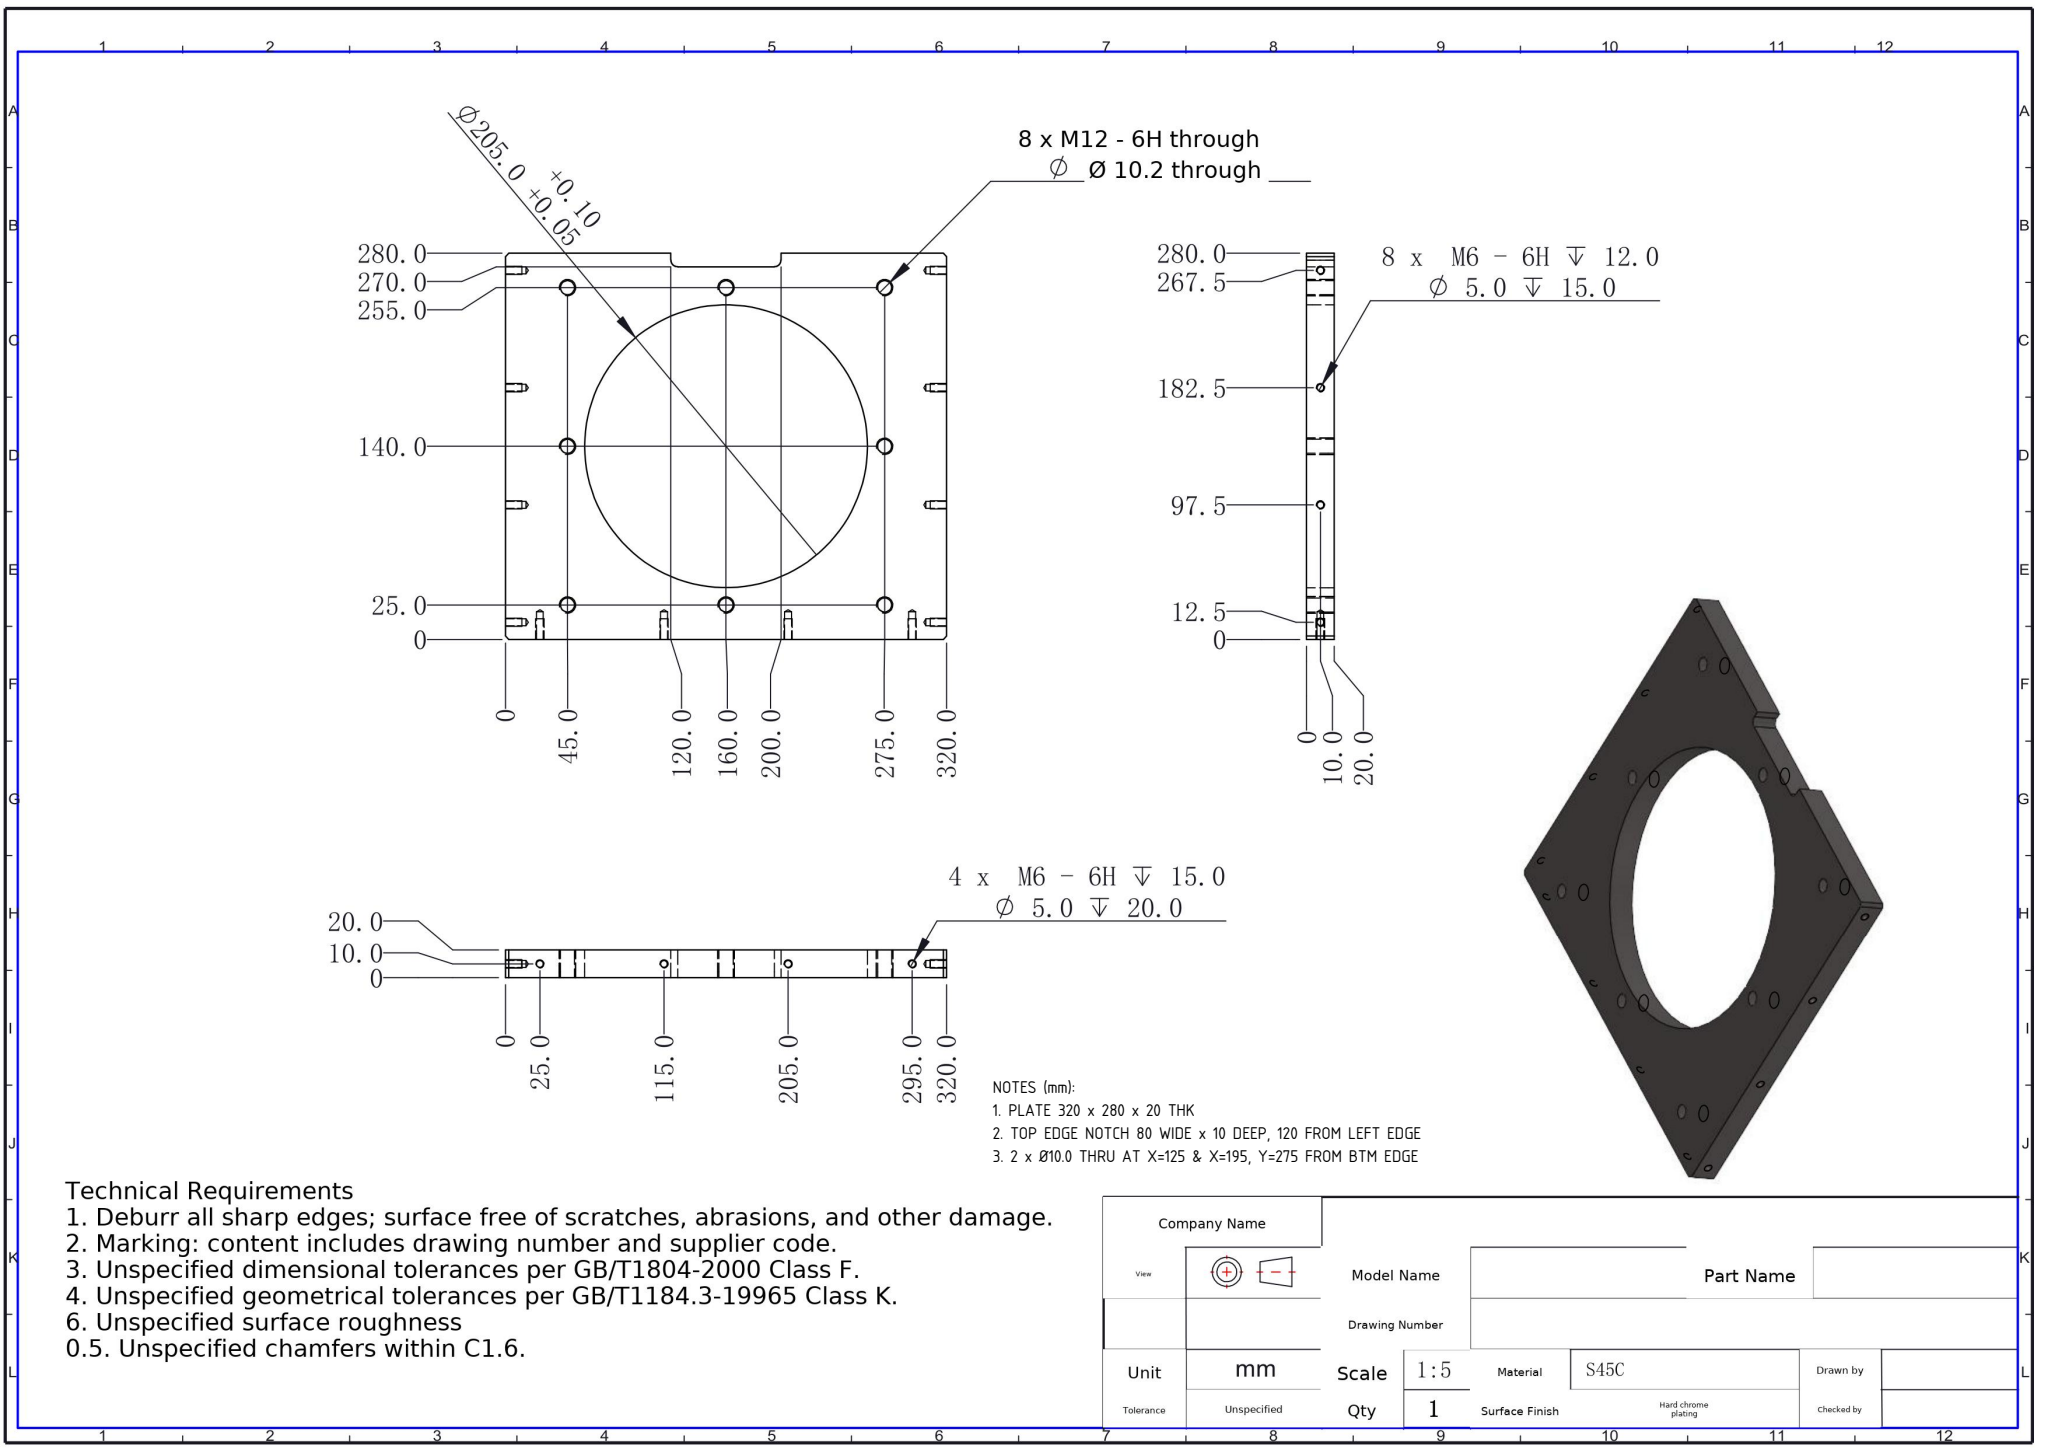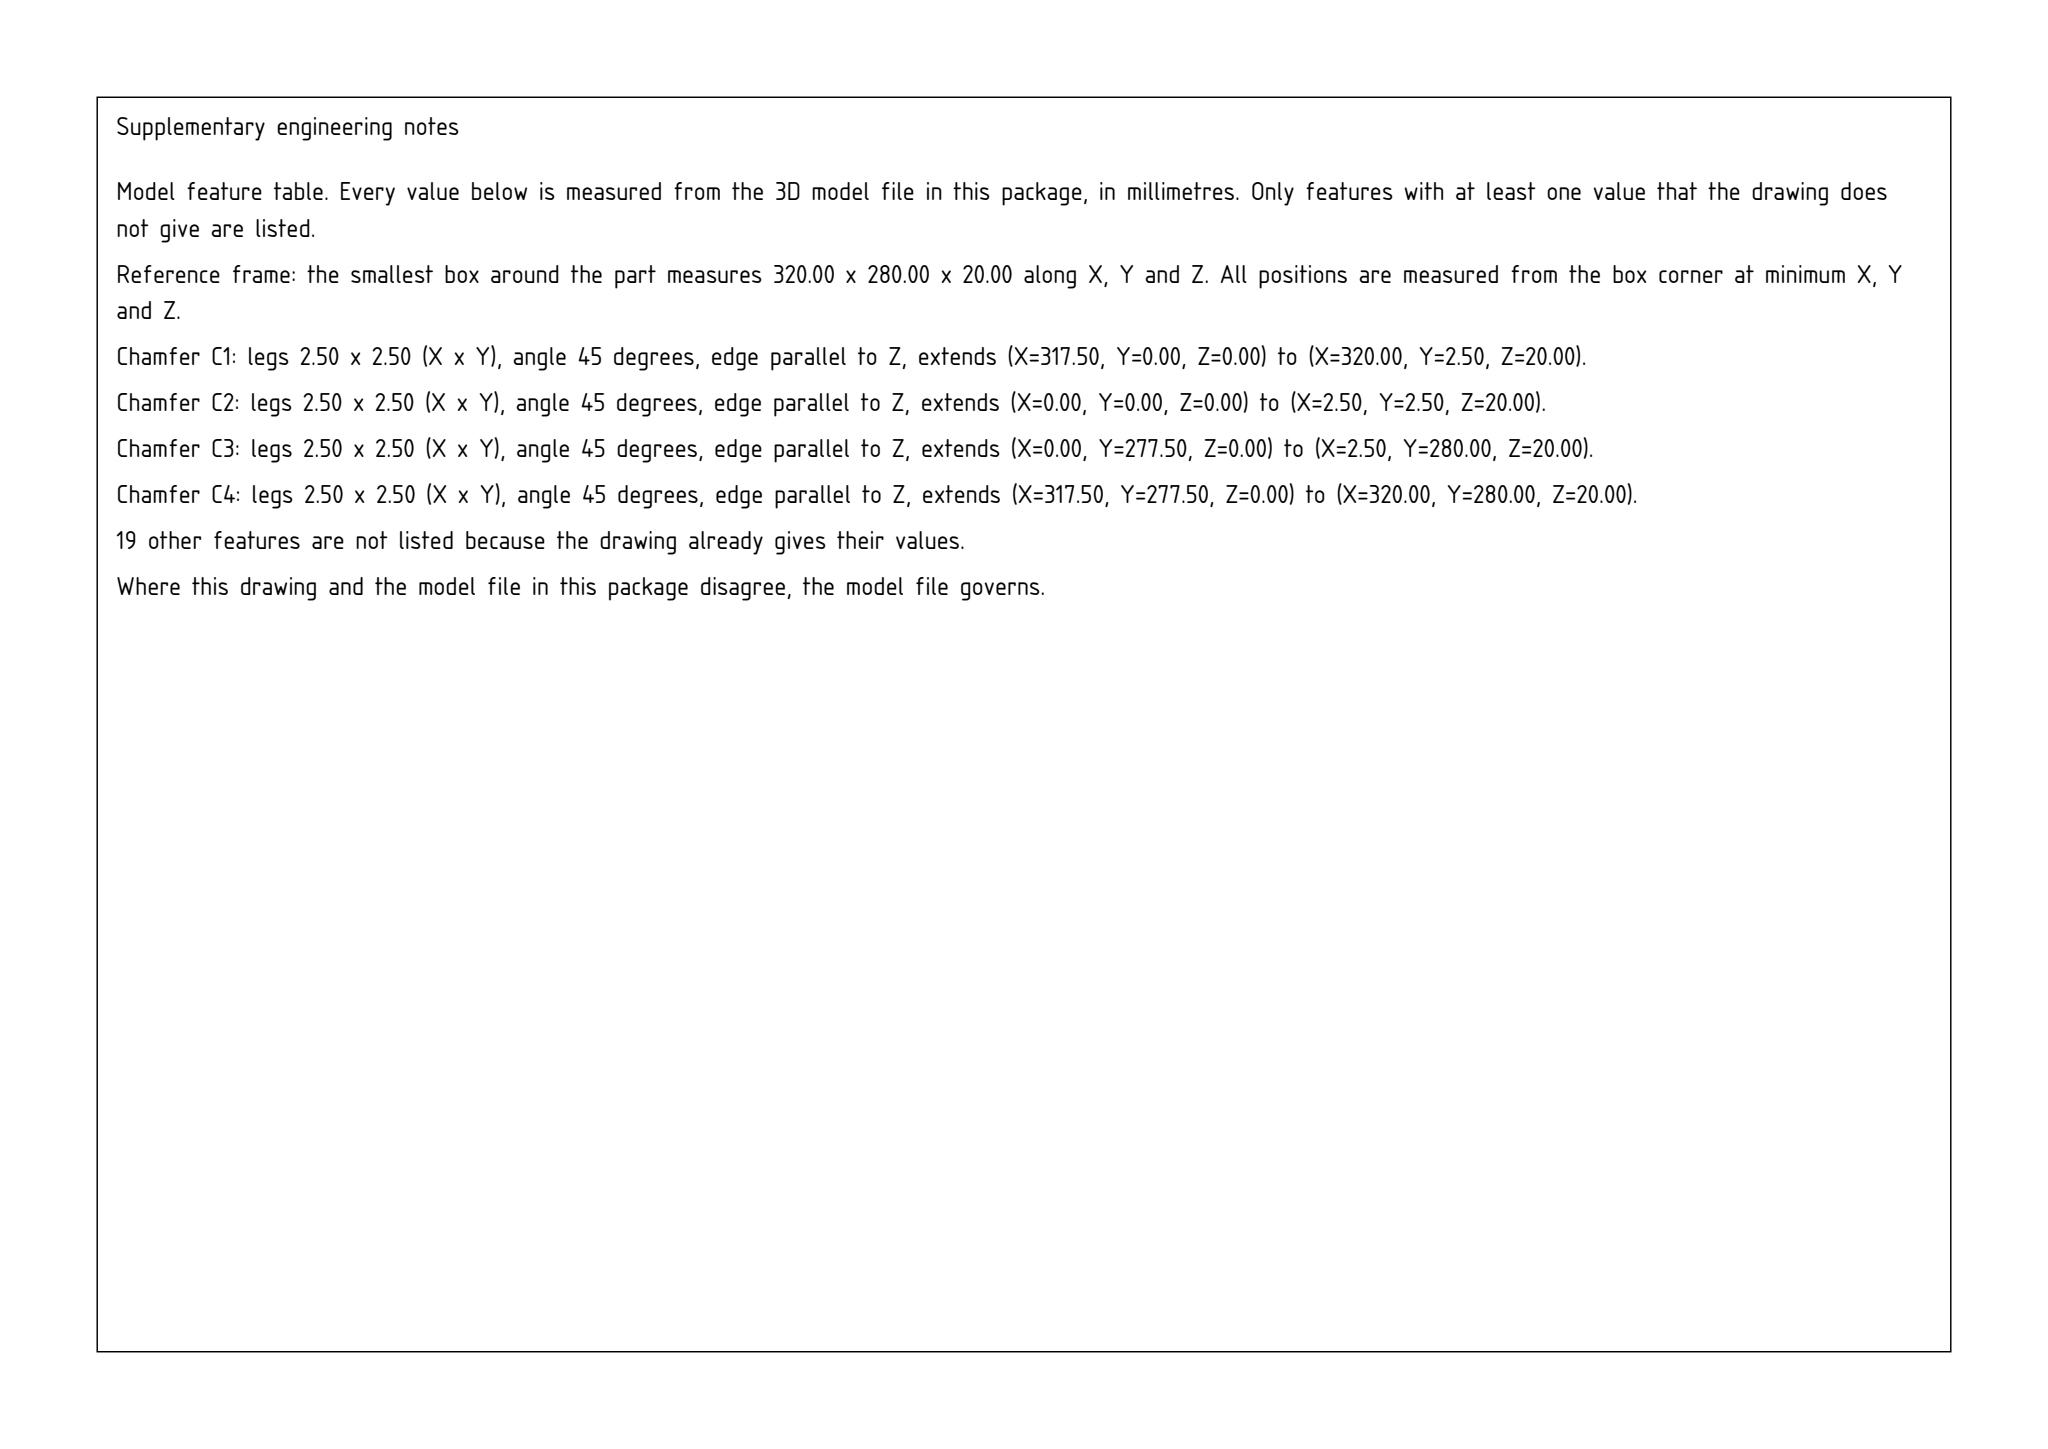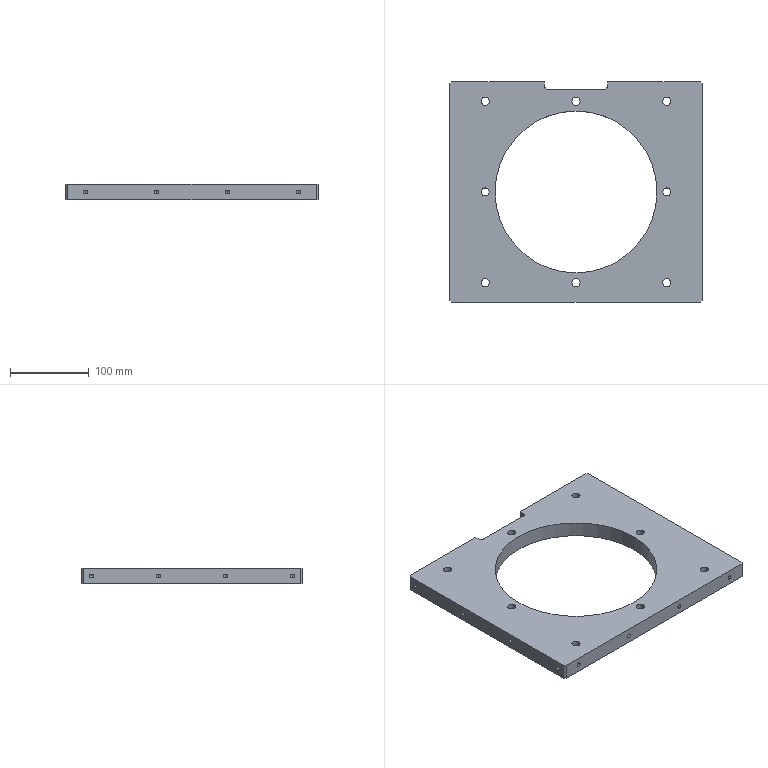Part | SolidWorks | mm | 1 solid | 82 faces | box 320 x 280 x 20 mm | volume 1098718 mm3 | cylinder 44 | cone 24 | plane 14 | commonest cylinder face diameters 5 x24 10.2 x16 205 x2 10 x2
Drawing notes:
PLATE 320 x 280 x 20 THK | from the solid: bbox_xyz 320.0 x 280.0 x 20.0
TOP EDGE NOTCH 80 WIDE x 10 DEEP, 120 FROM LEFT EDGE | from the solid: x planes 120.0 & 200.0 with y plane 270.0 vs top face y=280.0; 200-120=80, 280-270=10
2 x Ø10.0 THRU AT X=125 & X=195, Y=275 FROM BTM EDGE | from the solid: cylinders dia 10.0 axis z at (125,275) and (195,275), length 20 = full plate thk
build123d program:
from build123d import *

# Parameters (mm, degrees)
SKETCH1_R                  = 102.5
BOSS_EXTRUDE1_DEPTH        = 10
M6_TAPPED_HOLE1_AT_2_COUNT = 2
M6_TAPPED_HOLE1_AT_2_PITCH = 85
M6_TAPPED_HOLE1_AT_3_COUNT = 2
M6_TAPPED_HOLE1_AT_3_PITCH = 170
M6_TAPPED_HOLE1_AT_4_COUNT = 2
M6_TAPPED_HOLE1_AT_4_PITCH = 255
M12_TAPPED_HOLE1_D         = 10.2
M6_TAPPED_HOLE2_D          = 5
M6_TAPPED_HOLE2_DEPTH      = 20
M6_TAPPED_HOLE2_TIP        = 1.502
CHAMFER1_SIZE              = 2.5
FILLET1_R                  = 5


with BuildPart() as part:
    # Sketch1 → Boss-Extrude1 (new, symmetric)
    with BuildSketch(Plane.XY):
        Polygon((-160, 140), (-40, 140), (-40, 130), (40, 130), (40, 140), (160, 140), (160, -140), (-160, -140), align=None)
        Circle(SKETCH1_R, mode=Mode.SUBTRACT)
    extrude(amount=BOSS_EXTRUDE1_DEPTH, both=True)

    # Sketch3 → M6 Tapped Hole1 (revolve, cut)
    with BuildSketch(Plane(origin=(160, 127.5, 0), x_dir=(0, 0, -1), z_dir=(0, 1, 0))):
        Polygon((0, 0), (0, 16.502), (2.5, 15), (2.5, 0), align=None)
    m6_tapped_hole1 = revolve(axis=Axis((166.35, 127.5, 0), (-1, 0, 0)), mode=Mode.SUBTRACT)

    # M6 Tapped Hole1 at 2: M6 Tapped Hole1 ×2
    with Locations(*[(0, -i * M6_TAPPED_HOLE1_AT_2_PITCH, 0) for i in range(1, M6_TAPPED_HOLE1_AT_2_COUNT)]):
        add(m6_tapped_hole1, mode=Mode.SUBTRACT)

    # M6 Tapped Hole1 at 3: M6 Tapped Hole1 ×2
    with Locations(*[(0, -i * M6_TAPPED_HOLE1_AT_3_PITCH, 0) for i in range(1, M6_TAPPED_HOLE1_AT_3_COUNT)]):
        add(m6_tapped_hole1, mode=Mode.SUBTRACT)

    # M6 Tapped Hole1 at 4: M6 Tapped Hole1 ×2
    with Locations(*[(0, -i * M6_TAPPED_HOLE1_AT_4_PITCH, 0) for i in range(1, M6_TAPPED_HOLE1_AT_4_COUNT)]):
        add(m6_tapped_hole1, mode=Mode.SUBTRACT)

    # Mirror1: M6 Tapped Hole1 across plane
    add(m6_tapped_hole1.mirror(Plane(origin=(0, 0, 0), x_dir=(0, 0, 1), z_dir=(1, 0, 0))), mode=Mode.SUBTRACT)

    # Mirror1 copy 1 sketch → Mirror1 copy 1 (revolve, cut)
    with BuildSketch(Plane(origin=(-160, 42.5, 0), x_dir=(0, 0, -1), z_dir=(0, 1, 0))):
        Polygon((0, 0), (0, -16.502), (2.5, -15), (2.5, 0), align=None)
    revolve(axis=Axis((-166.35, 42.5, 0), (-1, 0, 0)), mode=Mode.SUBTRACT)

    # Mirror1 copy 2 sketch → Mirror1 copy 2 (revolve, cut)
    with BuildSketch(Plane(origin=(-160, -42.5, 0), x_dir=(0, 0, -1), z_dir=(0, 1, 0))):
        Polygon((0, 0), (0, -16.502), (2.5, -15), (2.5, 0), align=None)
    revolve(axis=Axis((-166.35, -42.5, 0), (-1, 0, 0)), mode=Mode.SUBTRACT)

    # Mirror1 copy 3 sketch → Mirror1 copy 3 (revolve, cut)
    with BuildSketch(Plane(origin=(-160, -127.5, 0), x_dir=(0, 0, -1), z_dir=(0, 1, 0))):
        Polygon((0, 0), (0, -16.502), (2.5, -15), (2.5, 0), align=None)
    revolve(axis=Axis((-166.35, -127.5, 0), (-1, 0, 0)), mode=Mode.SUBTRACT)

    # M12 Tapped Hole1 (through all)
    with Locations(Plane.XY.offset(10)):
        with Locations((-115, 115), (-115, 0), (0, 115), (115, 115), (115, 0), (115, -115), (0, -115), (-115, -115)):
            Hole(M12_TAPPED_HOLE1_D / 2)

    # M6 Tapped Hole2
    with Locations(Plane(origin=(0, -140, 0), x_dir=(-1, 0, 0), z_dir=(0, -1, 0))):
        with Locations((-135, 0), (-45, 0), (45, 0), (135, 0)):
            Hole(M6_TAPPED_HOLE2_D / 2, depth=M6_TAPPED_HOLE2_DEPTH)
            with Locations((0, 0, -(M6_TAPPED_HOLE2_DEPTH + M6_TAPPED_HOLE2_TIP / 2))):  # 118° drill point
                Cone(0, M6_TAPPED_HOLE2_D / 2, M6_TAPPED_HOLE2_TIP, mode=Mode.SUBTRACT)

    # Chamfer1
    chamfer1_edges = [part.edges().sort_by_distance(p)[0] for p in [
        (-160, 140, 0),
        (160, 140, 0),
        (160, -140, 0),
        (-160, -140, 0),
    ]]
    chamfer(chamfer1_edges, length=CHAMFER1_SIZE)

    # Fillet1
    fillet1_edges = [part.edges().sort_by_distance(p)[0] for p in [
        (-40, 130, 0),
        (40, 130, 0),
    ]]
    fillet(fillet1_edges, radius=FILLET1_R)


solid = part.part